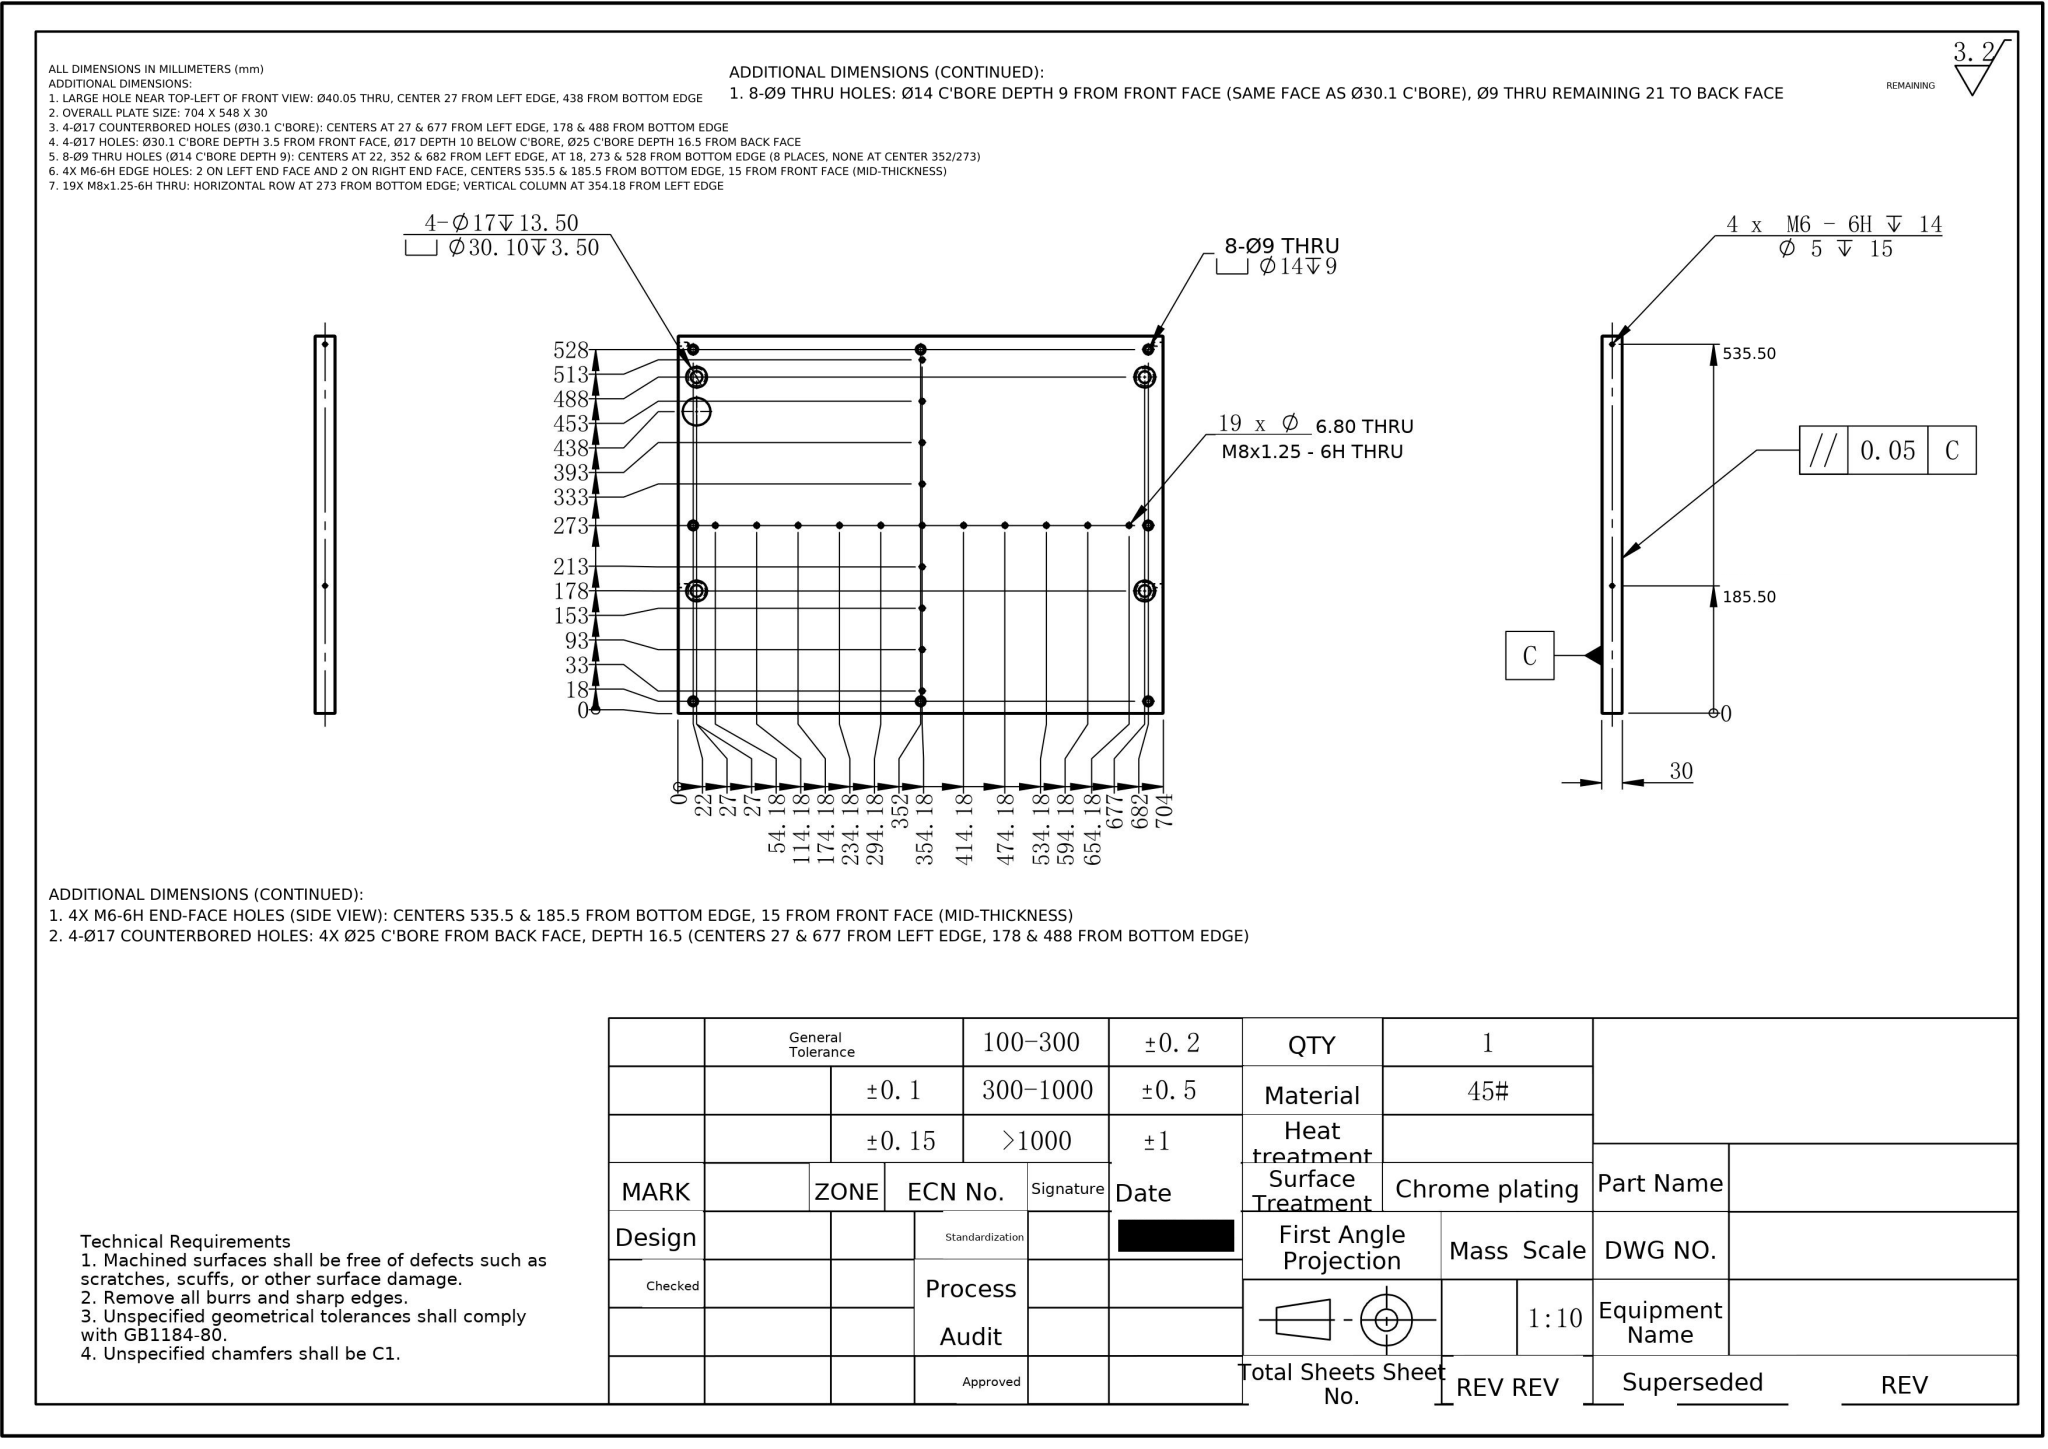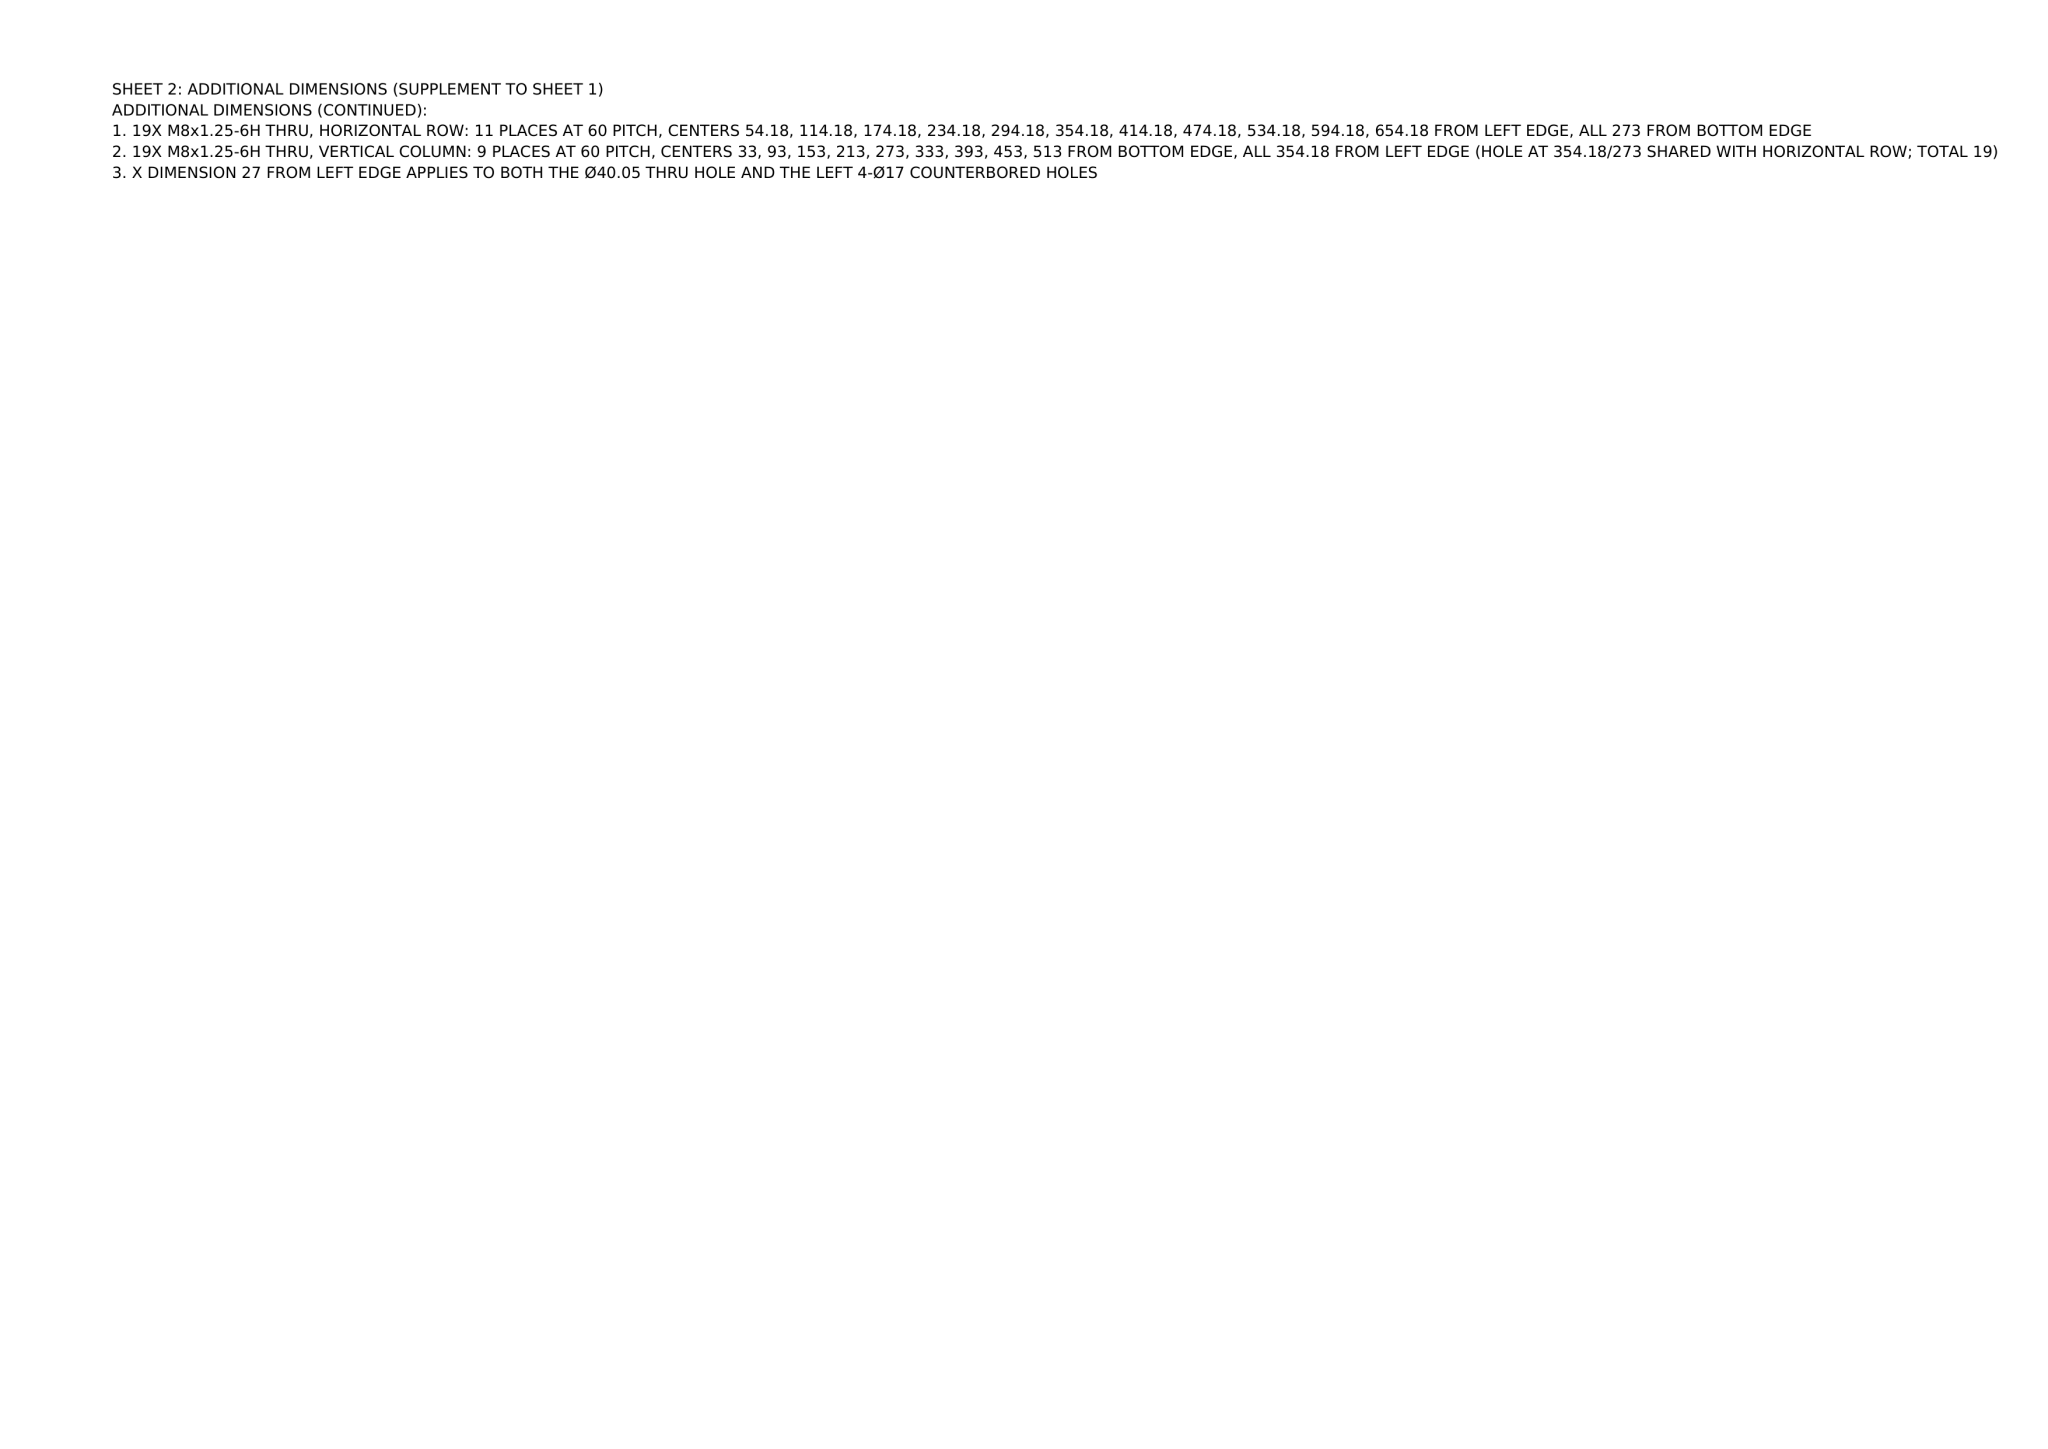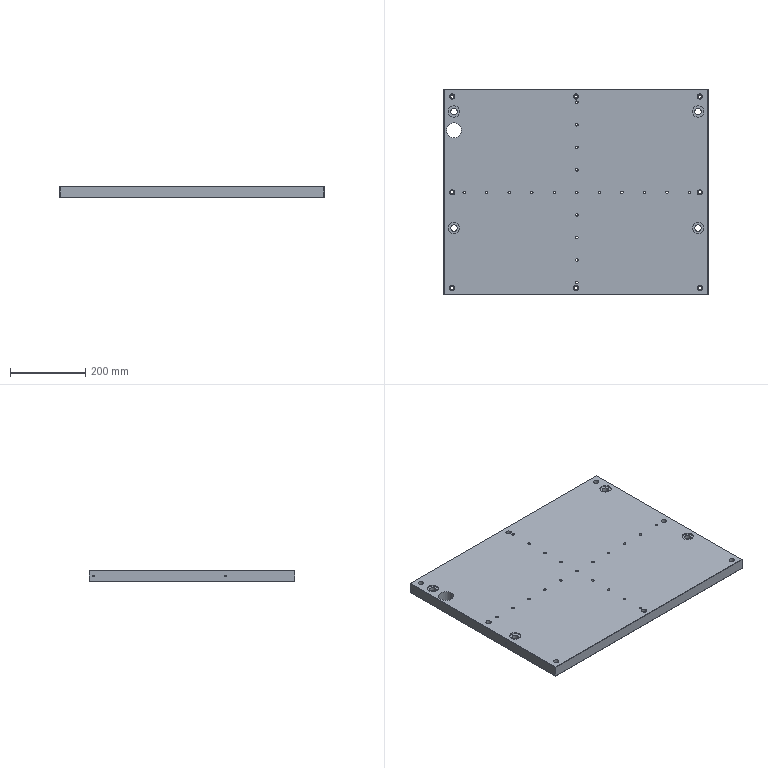Part | NX | mm | 1 solid | 150 faces | box 704 x 548 x 30 mm | volume 11438280 mm3 | cylinder 104 | plane 38 | cone 8 | commonest cylinder face diameters 6.8 x38 14 x16 9 x16 25 x8 30.1 x8 5 x8 17 x8 40.05 x2